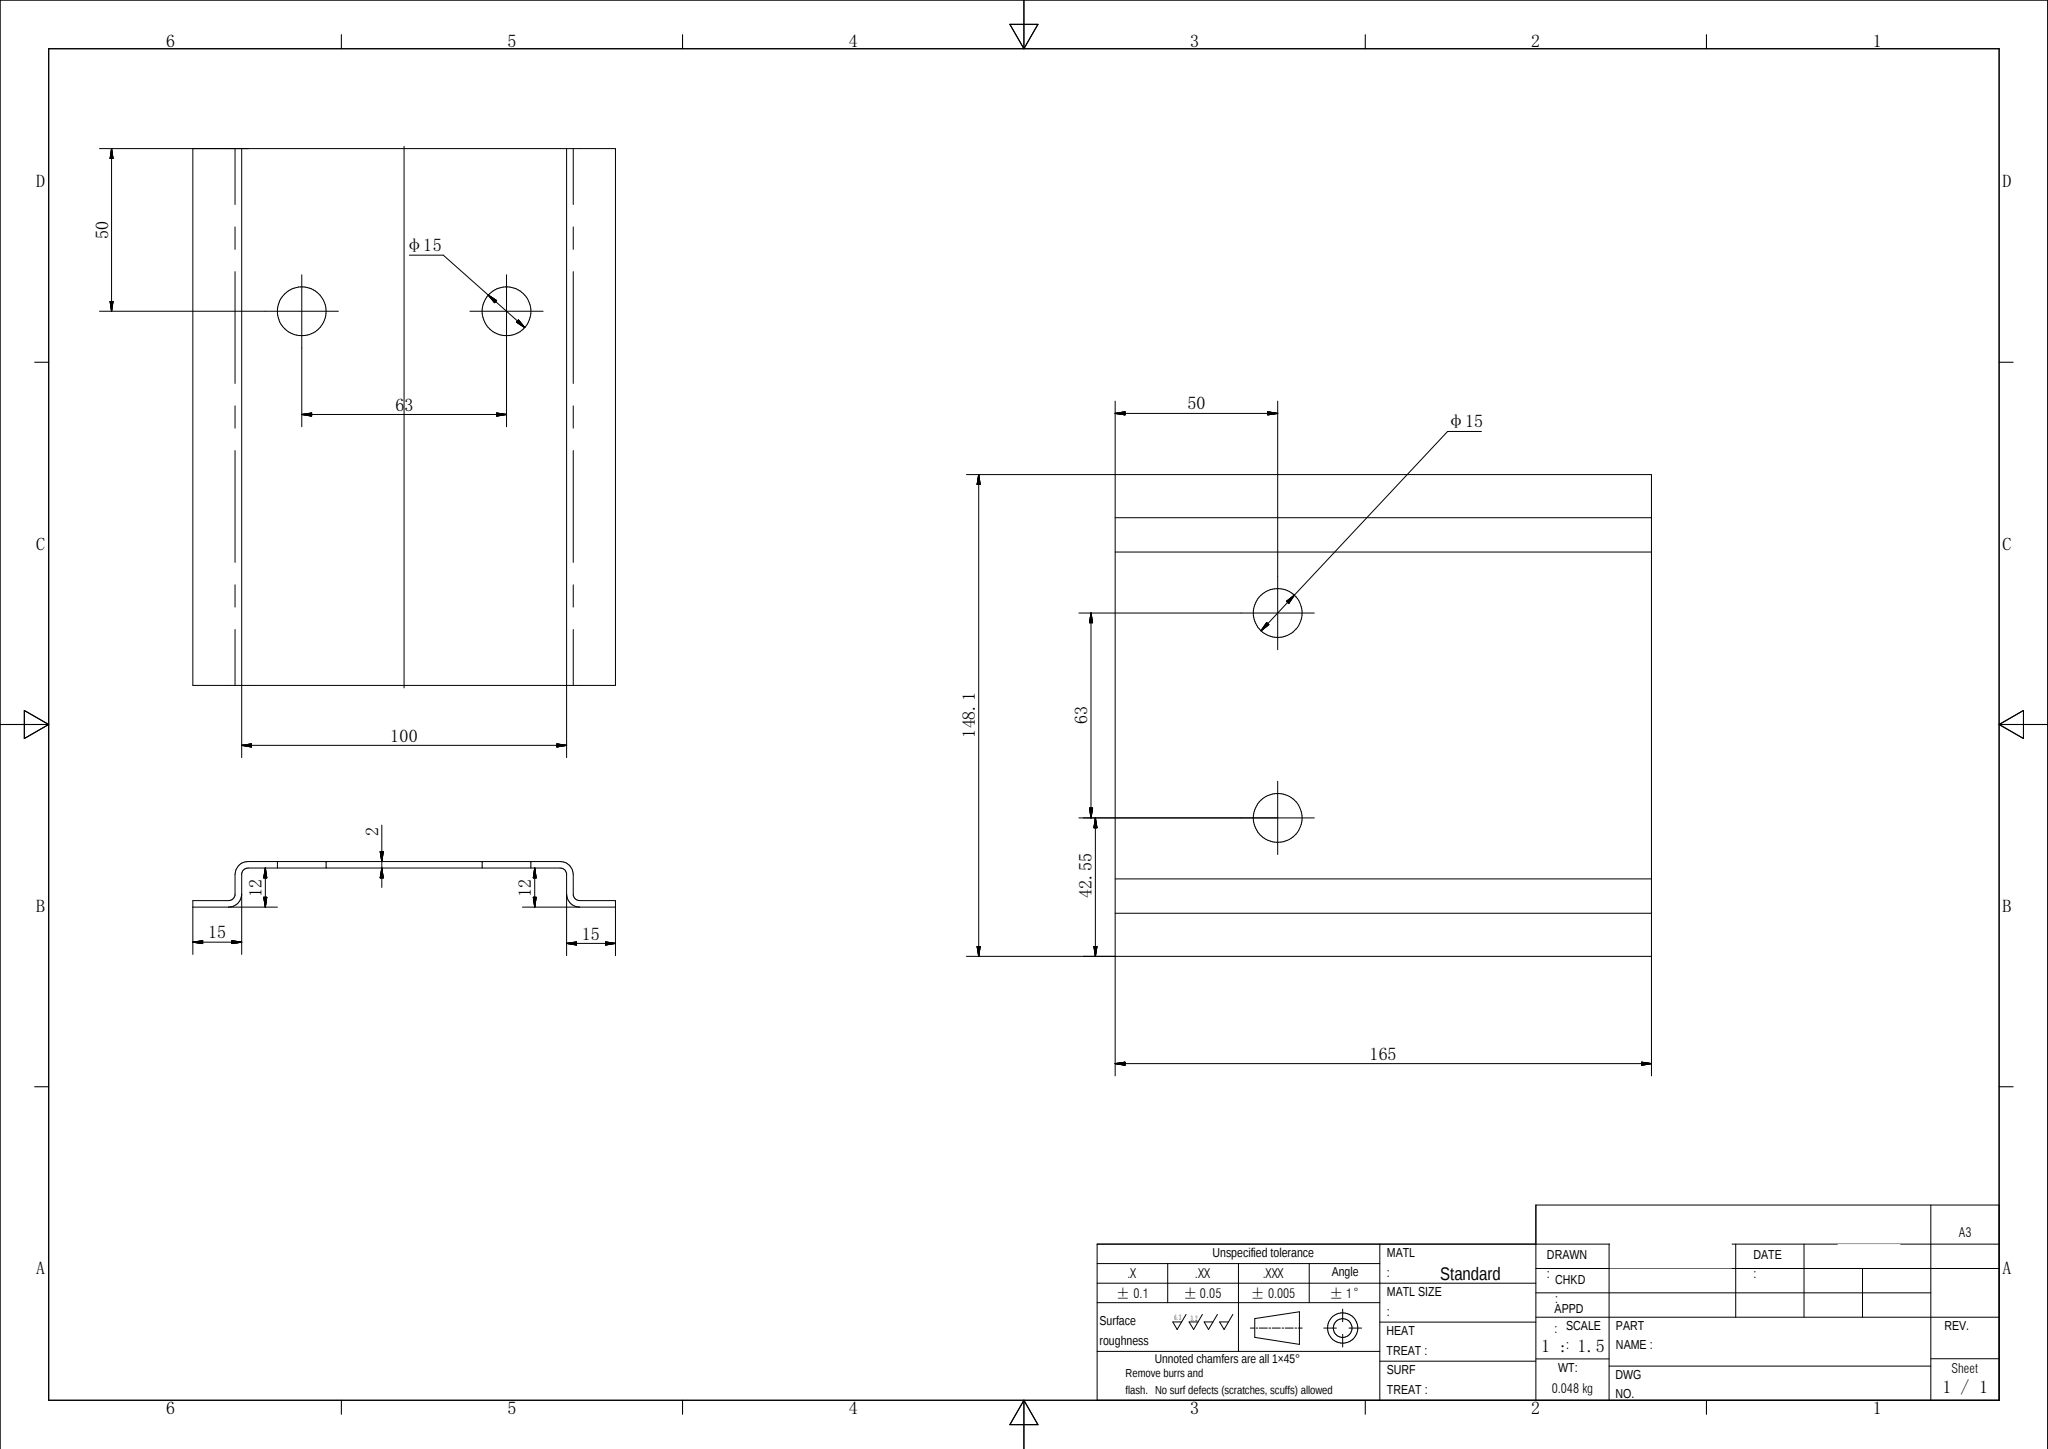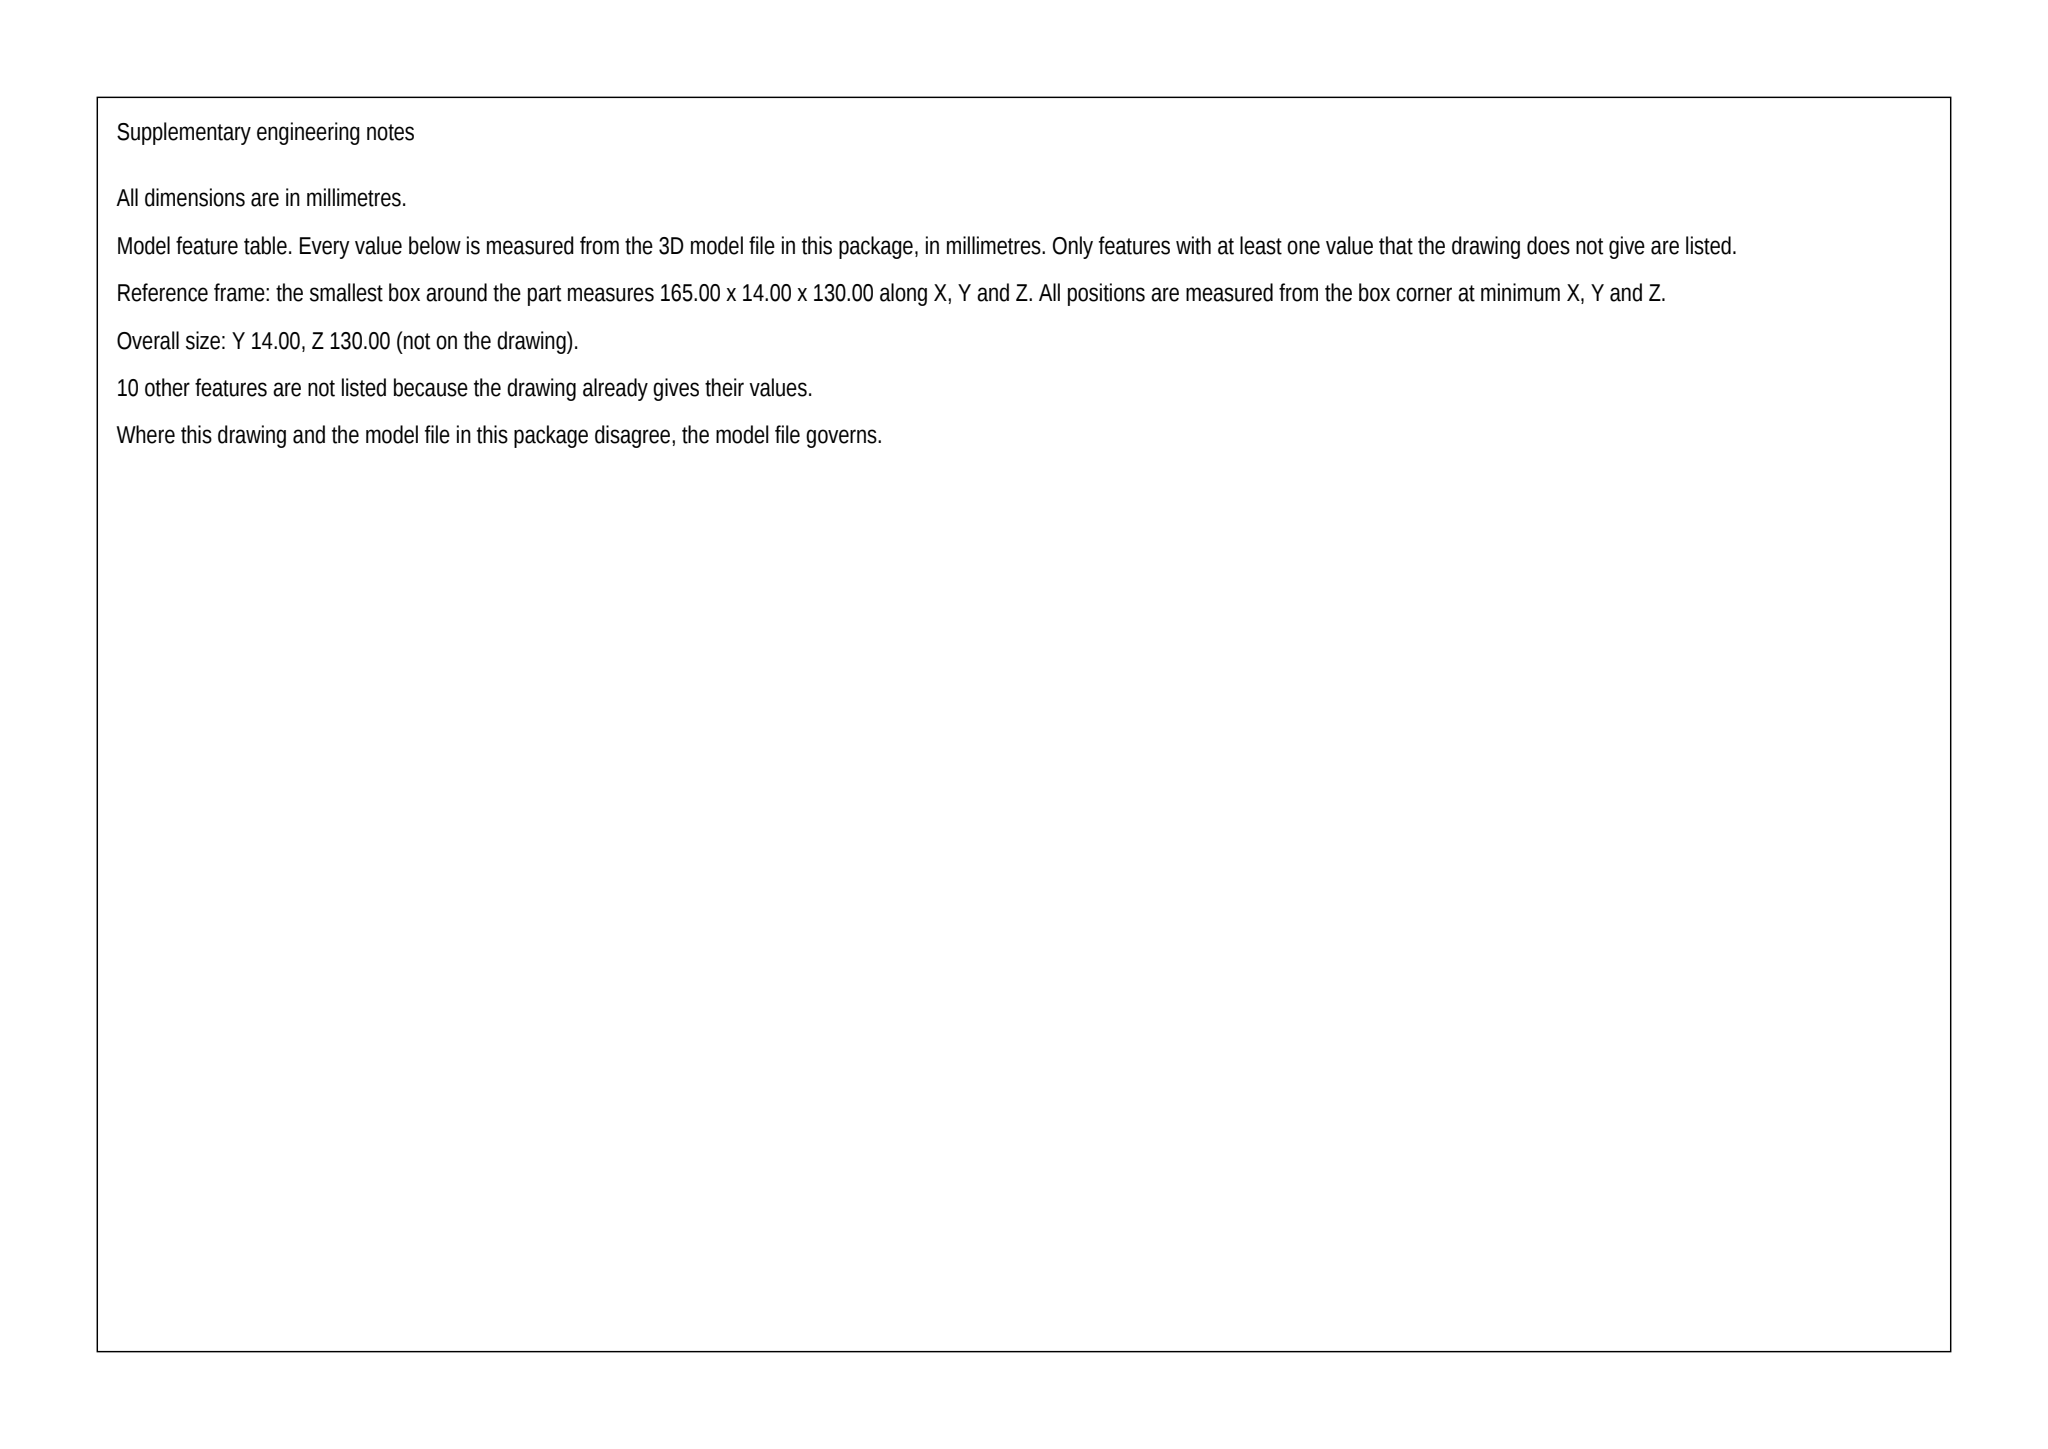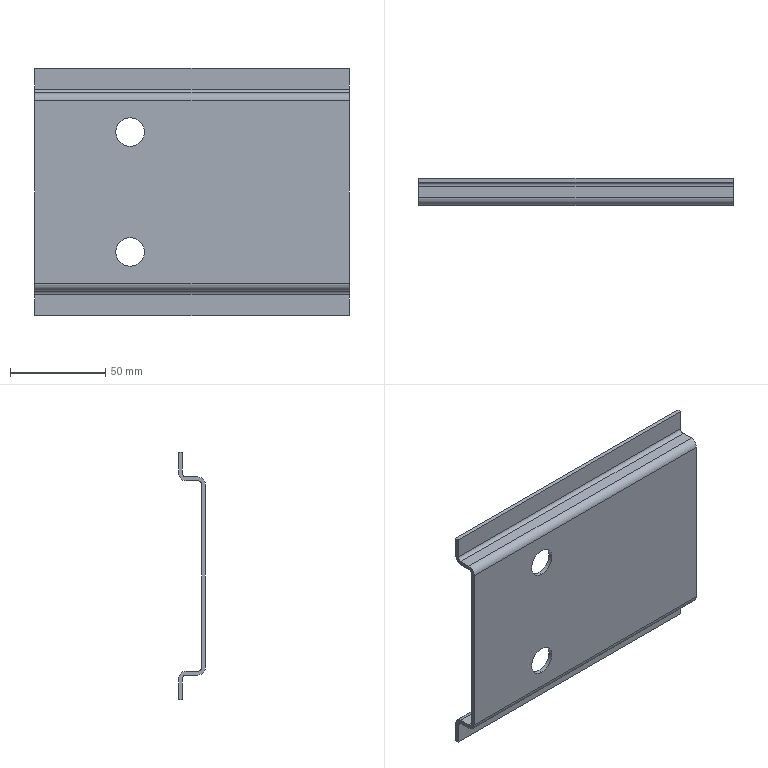Part | SolidWorks | mm | 1 solid | 26 faces | box 165 x 14 x 130 mm | volume 48413 mm3 | plane 14 | cylinder 12 | commonest cylinder face diameters 15 x4 4 x4 8 x4
Drawing notes:
ALL 4 BENDS: INSIDE R2, OUTSIDE R4 (THK 2) | from the solid: Cyl dia 4.0 (R2) and dia 8.0 (R4) along x at bend lines y=4/z=17,113 and y=10/z=11,119; plate planes y=0 & y=2 give THK 2
STEP:
#1=CARTESIAN_POINT('',(-32.5,0.,-39.));
#2=VERTEX_POINT('',#1);
#3=CARTESIAN_POINT('',(-32.5,0.,-24.));
#4=VERTEX_POINT('',#3);
#5=CARTESIAN_POINT('',(-32.5,0.,-31.5));
#6=DIRECTION('',(0.,1.,0.));
#7=DIRECTION('',(0.,0.,1.));
#8=AXIS2_PLACEMENT_3D('',#5,#6,#7);
#9=CIRCLE('',#8,7.5);
#10=EDGE_CURVE('',#2,#4,#9,.T.);
#11=ORIENTED_EDGE('',*,*,#10,.F.);
#12=CARTESIAN_POINT('',(-32.5,2.,-39.));
#13=VERTEX_POINT('',#12);
#14=CARTESIAN_POINT('',(-32.5,1.,-39.));
#15=DIRECTION('',(0.,1.,0.));
#16=VECTOR('',#15,1000.);
#17=LINE('',#14,#16);
#18=EDGE_CURVE('',#2,#13,#17,.T.);
#19=ORIENTED_EDGE('',*,*,#18,.T.);
#20=CARTESIAN_POINT('',(-32.5,2.,-24.));
#21=VERTEX_POINT('',#20);
#22=CARTESIAN_POINT('',(-32.5,2.,-31.5));
#23=DIRECTION('',(0.,-1.,0.));
#24=DIRECTION('',(0.,0.,1.));
#25=AXIS2_PLACEMENT_3D('',#22,#23,#24);
#26=CIRCLE('',#25,7.5);
#27=EDGE_CURVE('',#21,#13,#26,.T.);
#28=ORIENTED_EDGE('',*,*,#27,.F.);
#29=CARTESIAN_POINT('',(-32.5,1.,-24.));
#30=DIRECTION('',(0.,1.,0.));
#31=VECTOR('',#30,1000.);
#32=LINE('',#29,#31);
#33=EDGE_CURVE('',#4,#21,#32,.T.);
#34=ORIENTED_EDGE('',*,*,#33,.F.);
#35=EDGE_LOOP('',(#11,#19,#28,#34));
#36=FACE_OUTER_BOUND('',#35,.T.);
#37=CARTESIAN_POINT('',(-32.5,1.,-31.5));
#38=DIRECTION('',(0.,1.,0.));
#39=DIRECTION('',(0.,0.,1.));
#40=AXIS2_PLACEMENT_3D('',#37,#38,#39);
#41=CYLINDRICAL_SURFACE('',#40,7.5);
#42=ADVANCED_FACE('',(#36),#41,.F.);
#43=CARTESIAN_POINT('',(-32.5,0.,24.));
#44=VERTEX_POINT('',#43);
#45=CARTESIAN_POINT('',(-32.5,0.,39.));
#46=VERTEX_POINT('',#45);
#47=CARTESIAN_POINT('',(-32.5,0.,31.5));
#48=DIRECTION('',(0.,1.,0.));
#49=DIRECTION('',(0.,0.,1.));
#50=AXIS2_PLACEMENT_3D('',#47,#48,#49);
#51=CIRCLE('',#50,7.5);
#52=EDGE_CURVE('',#44,#46,#51,.T.);
#53=ORIENTED_EDGE('',*,*,#52,.F.);
#54=CARTESIAN_POINT('',(-32.5,2.,24.));
#55=VERTEX_POINT('',#54);
#56=CARTESIAN_POINT('',(-32.5,1.,24.));
#57=DIRECTION('',(0.,1.,0.));
#58=VECTOR('',#57,1000.);
#59=LINE('',#56,#58);
#60=EDGE_CURVE('',#44,#55,#59,.T.);
#61=ORIENTED_EDGE('',*,*,#60,.T.);
#62=CARTESIAN_POINT('',(-32.5,2.,39.));
#63=VERTEX_POINT('',#62);
#64=CARTESIAN_POINT('',(-32.5,2.,31.5));
#65=DIRECTION('',(0.,-1.,0.));
#66=DIRECTION('',(0.,0.,1.));
#67=AXIS2_PLACEMENT_3D('',#64,#65,#66);
#68=CIRCLE('',#67,7.5);
#69=EDGE_CURVE('',#63,#55,#68,.T.);
#70=ORIENTED_EDGE('',*,*,#69,.F.);
#71=CARTESIAN_POINT('',(-32.5,1.,39.));
#72=DIRECTION('',(0.,1.,0.));
#73=VECTOR('',#72,1000.);
#74=LINE('',#71,#73);
#75=EDGE_CURVE('',#46,#63,#74,.T.);
#76=ORIENTED_EDGE('',*,*,#75,.F.);
#77=EDGE_LOOP('',(#53,#61,#70,#76));
#78=FACE_OUTER_BOUND('',#77,.T.);
#79=CARTESIAN_POINT('',(-32.5,1.,31.5));
#80=DIRECTION('',(0.,1.,0.));
#81=DIRECTION('',(0.,0.,1.));
#82=AXIS2_PLACEMENT_3D('',#79,#80,#81);
#83=CYLINDRICAL_SURFACE('',#82,7.5);
#84=ADVANCED_FACE('',(#78),#83,.F.);
#85=ORIENTED_EDGE('',*,*,#27,.T.);
#86=CARTESIAN_POINT('',(-32.5,2.,-31.5));
#87=DIRECTION('',(0.,-1.,0.));
#88=DIRECTION('',(0.,0.,1.));
#89=AXIS2_PLACEMENT_3D('',#86,#87,#88);
#90=CIRCLE('',#89,7.5);
#91=EDGE_CURVE('',#13,#21,#90,.T.);
#92=ORIENTED_EDGE('',*,*,#91,.T.);
#93=EDGE_LOOP('',(#85,#92));
#94=FACE_BOUND('',#93,.T.);
#95=ORIENTED_EDGE('',*,*,#69,.T.);
#96=CARTESIAN_POINT('',(-32.5,2.,31.5));
#97=DIRECTION('',(0.,-1.,0.));
#98=DIRECTION('',(0.,0.,1.));
#99=AXIS2_PLACEMENT_3D('',#96,#97,#98);
#100=CIRCLE('',#99,7.5);
#101=EDGE_CURVE('',#55,#63,#100,.T.);
#102=ORIENTED_EDGE('',*,*,#101,.T.);
#103=EDGE_LOOP('',(#95,#102));
#104=FACE_BOUND('',#103,.T.);
#105=CARTESIAN_POINT('',(-82.5,2.,48.));
#106=VERTEX_POINT('',#105);
#107=CARTESIAN_POINT('',(82.5,2.,48.));
#108=VERTEX_POINT('',#107);
#109=CARTESIAN_POINT('',(-0.,2.,48.));
#110=DIRECTION('',(1.,0.,0.));
#111=VECTOR('',#110,1000.);
#112=LINE('',#109,#111);
#113=EDGE_CURVE('',#106,#108,#112,.T.);
#114=ORIENTED_EDGE('',*,*,#113,.T.);
#115=CARTESIAN_POINT('',(82.5,2.,-48.));
#116=VERTEX_POINT('',#115);
#117=CARTESIAN_POINT('',(82.5,2.,0.));
#118=DIRECTION('',(0.,0.,-1.));
#119=VECTOR('',#118,1000.);
#120=LINE('',#117,#119);
#121=EDGE_CURVE('',#108,#116,#120,.T.);
#122=ORIENTED_EDGE('',*,*,#121,.T.);
#123=CARTESIAN_POINT('',(-82.5,2.,-48.));
#124=VERTEX_POINT('',#123);
#125=CARTESIAN_POINT('',(-0.,2.,-48.));
#126=DIRECTION('',(-1.,0.,0.));
#127=VECTOR('',#126,1000.);
#128=LINE('',#125,#127);
#129=EDGE_CURVE('',#116,#124,#128,.T.);
#130=ORIENTED_EDGE('',*,*,#129,.T.);
#131=CARTESIAN_POINT('',(-82.5,2.,0.));
#132=DIRECTION('',(0.,0.,1.));
#133=VECTOR('',#132,1000.);
#134=LINE('',#131,#133);
#135=EDGE_CURVE('',#124,#106,#134,.T.);
#136=ORIENTED_EDGE('',*,*,#135,.T.);
#137=EDGE_LOOP('',(#114,#122,#130,#136));
#138=FACE_OUTER_BOUND('',#137,.T.);
#139=CARTESIAN_POINT('',(-0.,2.,0.));
#140=DIRECTION('',(0.,1.,0.));
#141=DIRECTION('',(0.,0.,1.));
#142=AXIS2_PLACEMENT_3D('',#139,#140,#141);
#143=PLANE('',#142);
#144=ADVANCED_FACE('',(#94,#104,#138),#143,.T.);
#145=ORIENTED_EDGE('',*,*,#18,.F.);
#146=CARTESIAN_POINT('',(-32.5,0.,-31.5));
#147=DIRECTION('',(0.,1.,0.));
#148=DIRECTION('',(0.,0.,1.));
#149=AXIS2_PLACEMENT_3D('',#146,#147,#148);
#150=CIRCLE('',#149,7.5);
#151=EDGE_CURVE('',#4,#2,#150,.T.);
#152=ORIENTED_EDGE('',*,*,#151,.F.);
#153=ORIENTED_EDGE('',*,*,#33,.T.);
#154=ORIENTED_EDGE('',*,*,#91,.F.);
#155=EDGE_LOOP('',(#145,#152,#153,#154));
#156=FACE_OUTER_BOUND('',#155,.T.);
#157=CARTESIAN_POINT('',(-32.5,1.,-31.5));
#158=DIRECTION('',(0.,1.,0.));
#159=DIRECTION('',(0.,0.,1.));
#160=AXIS2_PLACEMENT_3D('',#157,#158,#159);
#161=CYLINDRICAL_SURFACE('',#160,7.5);
#162=ADVANCED_FACE('',(#156),#161,.F.);
#163=ORIENTED_EDGE('',*,*,#60,.F.);
#164=CARTESIAN_POINT('',(-32.5,0.,31.5));
#165=DIRECTION('',(0.,1.,0.));
#166=DIRECTION('',(0.,0.,1.));
#167=AXIS2_PLACEMENT_3D('',#164,#165,#166);
#168=CIRCLE('',#167,7.5);
#169=EDGE_CURVE('',#46,#44,#168,.T.);
#170=ORIENTED_EDGE('',*,*,#169,.F.);
#171=ORIENTED_EDGE('',*,*,#75,.T.);
#172=ORIENTED_EDGE('',*,*,#101,.F.);
#173=EDGE_LOOP('',(#163,#170,#171,#172));
#174=FACE_OUTER_BOUND('',#173,.T.);
#175=CARTESIAN_POINT('',(-32.5,1.,31.5));
#176=DIRECTION('',(0.,1.,0.));
#177=DIRECTION('',(0.,0.,1.));
#178=AXIS2_PLACEMENT_3D('',#175,#176,#177);
#179=CYLINDRICAL_SURFACE('',#178,7.5);
#180=ADVANCED_FACE('',(#174),#179,.F.);
#181=ORIENTED_EDGE('',*,*,#121,.F.);
#182=CARTESIAN_POINT('',(82.5,4.,50.));
#183=VERTEX_POINT('',#182);
#184=CARTESIAN_POINT('',(82.5,4.,48.));
#185=DIRECTION('',(-1.,0.,0.));
#186=DIRECTION('',(0.,0.,1.));
#187=AXIS2_PLACEMENT_3D('',#184,#185,#186);
#188=CIRCLE('',#187,2.);
#189=EDGE_CURVE('',#108,#183,#188,.T.);
#190=ORIENTED_EDGE('',*,*,#189,.T.);
#191=CARTESIAN_POINT('',(82.5,10.,50.));
#192=VERTEX_POINT('',#191);
#193=CARTESIAN_POINT('',(82.5,6.738,50.));
#194=DIRECTION('',(0.,-1.,-0.));
#195=VECTOR('',#194,1000.);
#196=LINE('',#193,#195);
#197=EDGE_CURVE('',#192,#183,#196,.T.);
#198=ORIENTED_EDGE('',*,*,#197,.F.);
#199=CARTESIAN_POINT('',(82.5,14.,54.));
#200=VERTEX_POINT('',#199);
#201=CARTESIAN_POINT('',(82.5,10.,54.));
#202=DIRECTION('',(-1.,0.,0.));
#203=DIRECTION('',(0.,-0.,-1.));
#204=AXIS2_PLACEMENT_3D('',#201,#202,#203);
#205=CIRCLE('',#204,4.);
#206=EDGE_CURVE('',#200,#192,#205,.T.);
#207=ORIENTED_EDGE('',*,*,#206,.F.);
#208=CARTESIAN_POINT('',(82.5,14.,65.));
#209=VERTEX_POINT('',#208);
#210=CARTESIAN_POINT('',(82.5,14.,57.238));
#211=DIRECTION('',(0.,-0.,1.));
#212=VECTOR('',#211,1000.);
#213=LINE('',#210,#212);
#214=EDGE_CURVE('',#200,#209,#213,.T.);
#215=ORIENTED_EDGE('',*,*,#214,.T.);
#216=CARTESIAN_POINT('',(82.5,12.,65.));
#217=VERTEX_POINT('',#216);
#218=CARTESIAN_POINT('',(82.5,12.,65.));
#219=DIRECTION('',(-0.,-1.,0.));
#220=VECTOR('',#219,1000.);
#221=LINE('',#218,#220);
#222=EDGE_CURVE('',#209,#217,#221,.T.);
#223=ORIENTED_EDGE('',*,*,#222,.T.);
#224=CARTESIAN_POINT('',(82.5,12.,54.));
#225=VERTEX_POINT('',#224);
#226=CARTESIAN_POINT('',(82.5,12.,54.));
#227=DIRECTION('',(0.,-0.,-1.));
#228=VECTOR('',#227,1000.);
#229=LINE('',#226,#228);
#230=EDGE_CURVE('',#217,#225,#229,.T.);
#231=ORIENTED_EDGE('',*,*,#230,.T.);
#232=CARTESIAN_POINT('',(82.5,10.,52.));
#233=VERTEX_POINT('',#232);
#234=CARTESIAN_POINT('',(82.5,10.,54.));
#235=DIRECTION('',(-1.,0.,0.));
#236=DIRECTION('',(0.,-0.,-1.));
#237=AXIS2_PLACEMENT_3D('',#234,#235,#236);
#238=CIRCLE('',#237,2.);
#239=EDGE_CURVE('',#225,#233,#238,.T.);
#240=ORIENTED_EDGE('',*,*,#239,.T.);
#241=CARTESIAN_POINT('',(82.5,4.,52.));
#242=VERTEX_POINT('',#241);
#243=CARTESIAN_POINT('',(82.5,4.,52.));
#244=DIRECTION('',(0.,-1.,-0.));
#245=VECTOR('',#244,1000.);
#246=LINE('',#243,#245);
#247=EDGE_CURVE('',#233,#242,#246,.T.);
#248=ORIENTED_EDGE('',*,*,#247,.T.);
#249=CARTESIAN_POINT('',(82.5,0.,48.));
#250=VERTEX_POINT('',#249);
#251=CARTESIAN_POINT('',(82.5,4.,48.));
#252=DIRECTION('',(1.,0.,-0.));
#253=DIRECTION('',(0.,-0.,1.));
#254=AXIS2_PLACEMENT_3D('',#251,#252,#253);
#255=CIRCLE('',#254,4.);
#256=EDGE_CURVE('',#242,#250,#255,.T.);
#257=ORIENTED_EDGE('',*,*,#256,.T.);
#258=CARTESIAN_POINT('',(82.5,0.,-48.));
#259=VERTEX_POINT('',#258);
#260=CARTESIAN_POINT('',(82.5,0.,-52.));
#261=DIRECTION('',(0.,0.,-1.));
#262=VECTOR('',#261,1000.);
#263=LINE('',#260,#262);
#264=EDGE_CURVE('',#250,#259,#263,.T.);
#265=ORIENTED_EDGE('',*,*,#264,.T.);
#266=CARTESIAN_POINT('',(82.5,4.,-52.));
#267=VERTEX_POINT('',#266);
#268=CARTESIAN_POINT('',(82.5,4.,-48.));
#269=DIRECTION('',(1.,0.,0.));
#270=DIRECTION('',(0.,0.,-1.));
#271=AXIS2_PLACEMENT_3D('',#268,#269,#270);
#272=CIRCLE('',#271,4.);
#273=EDGE_CURVE('',#259,#267,#272,.T.);
#274=ORIENTED_EDGE('',*,*,#273,.T.);
#275=CARTESIAN_POINT('',(82.5,10.,-52.));
#276=VERTEX_POINT('',#275);
#277=CARTESIAN_POINT('',(82.5,4.,-52.));
#278=DIRECTION('',(0.,1.,0.));
#279=VECTOR('',#278,1000.);
#280=LINE('',#277,#279);
#281=EDGE_CURVE('',#267,#276,#280,.T.);
#282=ORIENTED_EDGE('',*,*,#281,.T.);
#283=CARTESIAN_POINT('',(82.5,12.,-54.));
#284=VERTEX_POINT('',#283);
#285=CARTESIAN_POINT('',(82.5,10.,-54.));
#286=DIRECTION('',(-1.,0.,-0.));
#287=DIRECTION('',(0.,0.,1.));
#288=AXIS2_PLACEMENT_3D('',#285,#286,#287);
#289=CIRCLE('',#288,2.);
#290=EDGE_CURVE('',#276,#284,#289,.T.);
#291=ORIENTED_EDGE('',*,*,#290,.T.);
#292=CARTESIAN_POINT('',(82.5,12.,-65.));
#293=VERTEX_POINT('',#292);
#294=CARTESIAN_POINT('',(82.5,12.,-54.));
#295=DIRECTION('',(0.,-0.,-1.));
#296=VECTOR('',#295,1000.);
#297=LINE('',#294,#296);
#298=EDGE_CURVE('',#284,#293,#297,.T.);
#299=ORIENTED_EDGE('',*,*,#298,.T.);
#300=CARTESIAN_POINT('',(82.5,14.,-65.));
#301=VERTEX_POINT('',#300);
#302=CARTESIAN_POINT('',(82.5,12.,-65.));
#303=DIRECTION('',(0.,1.,0.));
#304=VECTOR('',#303,1000.);
#305=LINE('',#302,#304);
#306=EDGE_CURVE('',#293,#301,#305,.T.);
#307=ORIENTED_EDGE('',*,*,#306,.T.);
#308=CARTESIAN_POINT('',(82.5,14.,-54.));
#309=VERTEX_POINT('',#308);
#310=CARTESIAN_POINT('',(82.5,14.,-57.238));
#311=DIRECTION('',(0.,0.,-1.));
#312=VECTOR('',#311,1000.);
#313=LINE('',#310,#312);
#314=EDGE_CURVE('',#309,#301,#313,.T.);
#315=ORIENTED_EDGE('',*,*,#314,.F.);
#316=CARTESIAN_POINT('',(82.5,10.,-50.));
#317=VERTEX_POINT('',#316);
#318=CARTESIAN_POINT('',(82.5,10.,-54.));
#319=DIRECTION('',(-1.,0.,-0.));
#320=DIRECTION('',(0.,0.,1.));
#321=AXIS2_PLACEMENT_3D('',#318,#319,#320);
#322=CIRCLE('',#321,4.);
#323=EDGE_CURVE('',#317,#309,#322,.T.);
#324=ORIENTED_EDGE('',*,*,#323,.F.);
#325=CARTESIAN_POINT('',(82.5,4.,-50.));
#326=VERTEX_POINT('',#325);
#327=CARTESIAN_POINT('',(82.5,6.738,-50.));
#328=DIRECTION('',(0.,1.,0.));
#329=VECTOR('',#328,1000.);
#330=LINE('',#327,#329);
#331=EDGE_CURVE('',#326,#317,#330,.T.);
#332=ORIENTED_EDGE('',*,*,#331,.F.);
#333=CARTESIAN_POINT('',(82.5,4.,-48.));
#334=DIRECTION('',(-1.,0.,0.));
#335=DIRECTION('',(0.,0.,-1.));
#336=AXIS2_PLACEMENT_3D('',#333,#334,#335);
#337=CIRCLE('',#336,2.);
#338=EDGE_CURVE('',#326,#116,#337,.T.);
#339=ORIENTED_EDGE('',*,*,#338,.T.);
#340=EDGE_LOOP('',(#181,#190,#198,#207,#215,#223,#231,#240,#248,#257,#265,#274,#282,#291,#299,#307,#315,#324,#332,#339));
#341=FACE_OUTER_BOUND('',#340,.T.);
#342=CARTESIAN_POINT('',(82.5,0.,-52.));
#343=DIRECTION('',(1.,0.,0.));
#344=DIRECTION('',(0.,0.,-1.));
#345=AXIS2_PLACEMENT_3D('',#342,#343,#344);
#346=PLANE('',#345);
#347=ADVANCED_FACE('',(#341),#346,.T.);
#348=ORIENTED_EDGE('',*,*,#189,.F.);
#349=ORIENTED_EDGE('',*,*,#113,.F.);
#350=CARTESIAN_POINT('',(-82.5,4.,50.));
#351=VERTEX_POINT('',#350);
#352=CARTESIAN_POINT('',(-82.5,4.,48.));
#353=DIRECTION('',(1.,0.,-0.));
#354=DIRECTION('',(0.,-0.,1.));
#355=AXIS2_PLACEMENT_3D('',#352,#353,#354);
#356=CIRCLE('',#355,2.);
#357=EDGE_CURVE('',#351,#106,#356,.T.);
#358=ORIENTED_EDGE('',*,*,#357,.F.);
#359=CARTESIAN_POINT('',(0.,4.,50.));
#360=DIRECTION('',(-1.,0.,0.));
#361=VECTOR('',#360,1000.);
#362=LINE('',#359,#361);
#363=EDGE_CURVE('',#183,#351,#362,.T.);
#364=ORIENTED_EDGE('',*,*,#363,.F.);
#365=EDGE_LOOP('',(#348,#349,#358,#364));
#366=FACE_OUTER_BOUND('',#365,.T.);
#367=CARTESIAN_POINT('',(0.,4.,48.));
#368=DIRECTION('',(-1.,0.,0.));
#369=DIRECTION('',(0.,0.,1.));
#370=AXIS2_PLACEMENT_3D('',#367,#368,#369);
#371=CYLINDRICAL_SURFACE('',#370,2.);
#372=ADVANCED_FACE('',(#366),#371,.F.);
#373=CARTESIAN_POINT('',(-82.5,0.,-48.));
#374=VERTEX_POINT('',#373);
#375=CARTESIAN_POINT('',(-82.5,0.,48.));
#376=VERTEX_POINT('',#375);
#377=CARTESIAN_POINT('',(-82.5,0.,52.));
#378=DIRECTION('',(0.,0.,1.));
#379=VECTOR('',#378,1000.);
#380=LINE('',#377,#379);
#381=EDGE_CURVE('',#374,#376,#380,.T.);
#382=ORIENTED_EDGE('',*,*,#381,.T.);
#383=CARTESIAN_POINT('',(-82.5,4.,52.));
#384=VERTEX_POINT('',#383);
#385=CARTESIAN_POINT('',(-82.5,4.,48.));
#386=DIRECTION('',(-1.,0.,0.));
#387=DIRECTION('',(0.,0.,1.));
#388=AXIS2_PLACEMENT_3D('',#385,#386,#387);
#389=CIRCLE('',#388,4.);
#390=EDGE_CURVE('',#376,#384,#389,.T.);
#391=ORIENTED_EDGE('',*,*,#390,.T.);
#392=CARTESIAN_POINT('',(-82.5,10.,52.));
#393=VERTEX_POINT('',#392);
#394=CARTESIAN_POINT('',(-82.5,4.,52.));
#395=DIRECTION('',(0.,1.,0.));
#396=VECTOR('',#395,1000.);
#397=LINE('',#394,#396);
#398=EDGE_CURVE('',#384,#393,#397,.T.);
#399=ORIENTED_EDGE('',*,*,#398,.T.);
#400=CARTESIAN_POINT('',(-82.5,12.,54.));
#401=VERTEX_POINT('',#400);
#402=CARTESIAN_POINT('',(-82.5,10.,54.));
#403=DIRECTION('',(1.,-0.,-0.));
#404=DIRECTION('',(0.,0.,-1.));
#405=AXIS2_PLACEMENT_3D('',#402,#403,#404);
#406=CIRCLE('',#405,2.);
#407=EDGE_CURVE('',#393,#401,#406,.T.);
#408=ORIENTED_EDGE('',*,*,#407,.T.);
#409=CARTESIAN_POINT('',(-82.5,12.,65.));
#410=VERTEX_POINT('',#409);
#411=CARTESIAN_POINT('',(-82.5,12.,54.));
#412=DIRECTION('',(0.,0.,1.));
#413=VECTOR('',#412,1000.);
#414=LINE('',#411,#413);
#415=EDGE_CURVE('',#401,#410,#414,.T.);
#416=ORIENTED_EDGE('',*,*,#415,.T.);
#417=CARTESIAN_POINT('',(-82.5,14.,65.));
#418=VERTEX_POINT('',#417);
#419=CARTESIAN_POINT('',(-82.5,12.,65.));
#420=DIRECTION('',(0.,1.,-0.));
#421=VECTOR('',#420,1000.);
#422=LINE('',#419,#421);
#423=EDGE_CURVE('',#410,#418,#422,.T.);
#424=ORIENTED_EDGE('',*,*,#423,.T.);
#425=CARTESIAN_POINT('',(-82.5,14.,54.));
#426=VERTEX_POINT('',#425);
#427=CARTESIAN_POINT('',(-82.5,14.,57.238));
#428=DIRECTION('',(0.,0.,-1.));
#429=VECTOR('',#428,1000.);
#430=LINE('',#427,#429);
#431=EDGE_CURVE('',#418,#426,#430,.T.);
#432=ORIENTED_EDGE('',*,*,#431,.T.);
#433=CARTESIAN_POINT('',(-82.5,10.,50.));
#434=VERTEX_POINT('',#433);
#435=CARTESIAN_POINT('',(-82.5,10.,54.));
#436=DIRECTION('',(1.,-0.,-0.));
#437=DIRECTION('',(0.,0.,-1.));
#438=AXIS2_PLACEMENT_3D('',#435,#436,#437);
#439=CIRCLE('',#438,4.);
#440=EDGE_CURVE('',#434,#426,#439,.T.);
#441=ORIENTED_EDGE('',*,*,#440,.F.);
#442=CARTESIAN_POINT('',(-82.5,6.738,50.));
#443=DIRECTION('',(0.,1.,0.));
#444=VECTOR('',#443,1000.);
#445=LINE('',#442,#444);
#446=EDGE_CURVE('',#351,#434,#445,.T.);
#447=ORIENTED_EDGE('',*,*,#446,.F.);
#448=ORIENTED_EDGE('',*,*,#357,.T.);
#449=ORIENTED_EDGE('',*,*,#135,.F.);
#450=CARTESIAN_POINT('',(-82.5,4.,-50.));
#451=VERTEX_POINT('',#450);
#452=CARTESIAN_POINT('',(-82.5,4.,-48.));
#453=DIRECTION('',(1.,0.,0.));
#454=DIRECTION('',(0.,0.,-1.));
#455=AXIS2_PLACEMENT_3D('',#452,#453,#454);
#456=CIRCLE('',#455,2.);
#457=EDGE_CURVE('',#124,#451,#456,.T.);
#458=ORIENTED_EDGE('',*,*,#457,.T.);
#459=CARTESIAN_POINT('',(-82.5,10.,-50.));
#460=VERTEX_POINT('',#459);
#461=CARTESIAN_POINT('',(-82.5,6.738,-50.));
#462=DIRECTION('',(0.,-1.,-0.));
#463=VECTOR('',#462,1000.);
#464=LINE('',#461,#463);
#465=EDGE_CURVE('',#460,#451,#464,.T.);
#466=ORIENTED_EDGE('',*,*,#465,.F.);
#467=CARTESIAN_POINT('',(-82.5,14.,-54.));
#468=VERTEX_POINT('',#467);
#469=CARTESIAN_POINT('',(-82.5,10.,-54.));
#470=DIRECTION('',(1.,-0.,0.));
#471=DIRECTION('',(0.,0.,1.));
#472=AXIS2_PLACEMENT_3D('',#469,#470,#471);
#473=CIRCLE('',#472,4.);
#474=EDGE_CURVE('',#468,#460,#473,.T.);
#475=ORIENTED_EDGE('',*,*,#474,.F.);
#476=CARTESIAN_POINT('',(-82.5,14.,-65.));
#477=VERTEX_POINT('',#476);
#478=CARTESIAN_POINT('',(-82.5,14.,-57.238));
#479=DIRECTION('',(0.,-0.,1.));
#480=VECTOR('',#479,1000.);
#481=LINE('',#478,#480);
#482=EDGE_CURVE('',#477,#468,#481,.T.);
#483=ORIENTED_EDGE('',*,*,#482,.F.);
#484=CARTESIAN_POINT('',(-82.5,12.,-65.));
#485=VERTEX_POINT('',#484);
#486=CARTESIAN_POINT('',(-82.5,12.,-65.));
#487=DIRECTION('',(-0.,-1.,0.));
#488=VECTOR('',#487,1000.);
#489=LINE('',#486,#488);
#490=EDGE_CURVE('',#477,#485,#489,.T.);
#491=ORIENTED_EDGE('',*,*,#490,.T.);
#492=CARTESIAN_POINT('',(-82.5,12.,-54.));
#493=VERTEX_POINT('',#492);
#494=CARTESIAN_POINT('',(-82.5,12.,-54.));
#495=DIRECTION('',(-0.,0.,1.));
#496=VECTOR('',#495,1000.);
#497=LINE('',#494,#496);
#498=EDGE_CURVE('',#485,#493,#497,.T.);
#499=ORIENTED_EDGE('',*,*,#498,.T.);
#500=CARTESIAN_POINT('',(-82.5,10.,-52.));
#501=VERTEX_POINT('',#500);
#502=CARTESIAN_POINT('',(-82.5,10.,-54.));
#503=DIRECTION('',(1.,-0.,0.));
#504=DIRECTION('',(0.,0.,1.));
#505=AXIS2_PLACEMENT_3D('',#502,#503,#504);
#506=CIRCLE('',#505,2.);
#507=EDGE_CURVE('',#493,#501,#506,.T.);
#508=ORIENTED_EDGE('',*,*,#507,.T.);
#509=CARTESIAN_POINT('',(-82.5,4.,-52.));
#510=VERTEX_POINT('',#509);
#511=CARTESIAN_POINT('',(-82.5,4.,-52.));
#512=DIRECTION('',(0.,-1.,0.));
#513=VECTOR('',#512,1000.);
#514=LINE('',#511,#513);
#515=EDGE_CURVE('',#501,#510,#514,.T.);
#516=ORIENTED_EDGE('',*,*,#515,.T.);
#517=CARTESIAN_POINT('',(-82.5,4.,-48.));
#518=DIRECTION('',(-1.,0.,0.));
#519=DIRECTION('',(0.,0.,-1.));
#520=AXIS2_PLACEMENT_3D('',#517,#518,#519);
#521=CIRCLE('',#520,4.);
#522=EDGE_CURVE('',#510,#374,#521,.T.);
#523=ORIENTED_EDGE('',*,*,#522,.T.);
#524=EDGE_LOOP('',(#382,#391,#399,#408,#416,#424,#432,#441,#447,#448,#449,#458,#466,#475,#483,#491,#499,#508,#516,#523));
#525=FACE_OUTER_BOUND('',#524,.T.);
#526=CARTESIAN_POINT('',(-82.5,0.,52.));
#527=DIRECTION('',(-1.,0.,0.));
#528=DIRECTION('',(0.,0.,1.));
#529=AXIS2_PLACEMENT_3D('',#526,#527,#528);
#530=PLANE('',#529);
#531=ADVANCED_FACE('',(#525),#530,.T.);
#532=ORIENTED_EDGE('',*,*,#457,.F.);
#533=ORIENTED_EDGE('',*,*,#129,.F.);
#534=ORIENTED_EDGE('',*,*,#338,.F.);
#535=CARTESIAN_POINT('',(0.,4.,-50.));
#536=DIRECTION('',(1.,0.,0.));
#537=VECTOR('',#536,1000.);
#538=LINE('',#535,#537);
#539=EDGE_CURVE('',#451,#326,#538,.T.);
#540=ORIENTED_EDGE('',*,*,#539,.F.);
#541=EDGE_LOOP('',(#532,#533,#534,#540));
#542=FACE_OUTER_BOUND('',#541,.T.);
#543=CARTESIAN_POINT('',(0.,4.,-48.));
#544=DIRECTION('',(1.,0.,0.));
#545=DIRECTION('',(0.,0.,-1.));
#546=AXIS2_PLACEMENT_3D('',#543,#544,#545);
#547=CYLINDRICAL_SURFACE('',#546,2.);
#548=ADVANCED_FACE('',(#542),#547,.F.);
#549=ORIENTED_EDGE('',*,*,#151,.T.);
#550=ORIENTED_EDGE('',*,*,#10,.T.);
#551=EDGE_LOOP('',(#549,#550));
#552=FACE_BOUND('',#551,.T.);
#553=ORIENTED_EDGE('',*,*,#169,.T.);
#554=ORIENTED_EDGE('',*,*,#52,.T.);
#555=EDGE_LOOP('',(#553,#554));
#556=FACE_BOUND('',#555,.T.);
#557=ORIENTED_EDGE('',*,*,#264,.F.);
#558=CARTESIAN_POINT('',(-0.,0.,48.));
#559=DIRECTION('',(1.,0.,0.));
#560=VECTOR('',#559,1000.);
#561=LINE('',#558,#560);
#562=EDGE_CURVE('',#376,#250,#561,.T.);
#563=ORIENTED_EDGE('',*,*,#562,.F.);
#564=ORIENTED_EDGE('',*,*,#381,.F.);
#565=CARTESIAN_POINT('',(-0.,0.,-48.));
#566=DIRECTION('',(-1.,0.,0.));
#567=VECTOR('',#566,1000.);
#568=LINE('',#565,#567);
#569=EDGE_CURVE('',#259,#374,#568,.T.);
#570=ORIENTED_EDGE('',*,*,#569,.F.);
#571=EDGE_LOOP('',(#557,#563,#564,#570));
#572=FACE_OUTER_BOUND('',#571,.T.);
#573=CARTESIAN_POINT('',(-0.,0.,0.));
#574=DIRECTION('',(0.,1.,0.));
#575=DIRECTION('',(0.,0.,1.));
#576=AXIS2_PLACEMENT_3D('',#573,#574,#575);
#577=PLANE('',#576);
#578=ADVANCED_FACE('',(#552,#556,#572),#577,.F.);
#579=ORIENTED_EDGE('',*,*,#363,.T.);
#580=ORIENTED_EDGE('',*,*,#446,.T.);
#581=CARTESIAN_POINT('',(-0.,10.,50.));
#582=DIRECTION('',(1.,0.,-0.));
#583=VECTOR('',#582,1000.);
#584=LINE('',#581,#583);
#585=EDGE_CURVE('',#434,#192,#584,.T.);
#586=ORIENTED_EDGE('',*,*,#585,.T.);
#587=ORIENTED_EDGE('',*,*,#197,.T.);
#588=EDGE_LOOP('',(#579,#580,#586,#587));
#589=FACE_OUTER_BOUND('',#588,.T.);
#590=CARTESIAN_POINT('',(-0.,6.738,50.));
#591=DIRECTION('',(-0.,0.,-1.));
#592=DIRECTION('',(0.,1.,0.));
#593=AXIS2_PLACEMENT_3D('',#590,#591,#592);
#594=PLANE('',#593);
#595=ADVANCED_FACE('',(#589),#594,.T.);
#596=ORIENTED_EDGE('',*,*,#539,.T.);
#597=ORIENTED_EDGE('',*,*,#331,.T.);
#598=CARTESIAN_POINT('',(0.,10.,-50.));
#599=DIRECTION('',(-1.,-0.,0.));
#600=VECTOR('',#599,1000.);
#601=LINE('',#598,#600);
#602=EDGE_CURVE('',#317,#460,#601,.T.);
#603=ORIENTED_EDGE('',*,*,#602,.T.);
#604=ORIENTED_EDGE('',*,*,#465,.T.);
#605=EDGE_LOOP('',(#596,#597,#603,#604));
#606=FACE_OUTER_BOUND('',#605,.T.);
#607=CARTESIAN_POINT('',(0.,6.738,-50.));
#608=DIRECTION('',(0.,-0.,1.));
#609=DIRECTION('',(0.,-1.,-0.));
#610=AXIS2_PLACEMENT_3D('',#607,#608,#609);
#611=PLANE('',#610);
#612=ADVANCED_FACE('',(#606),#611,.T.);
#613=ORIENTED_EDGE('',*,*,#569,.T.);
#614=ORIENTED_EDGE('',*,*,#522,.F.);
#615=CARTESIAN_POINT('',(0.,4.,-52.));
#616=DIRECTION('',(1.,0.,0.));
#617=VECTOR('',#616,1000.);
#618=LINE('',#615,#617);
#619=EDGE_CURVE('',#510,#267,#618,.T.);
#620=ORIENTED_EDGE('',*,*,#619,.T.);
#621=ORIENTED_EDGE('',*,*,#273,.F.);
#622=EDGE_LOOP('',(#613,#614,#620,#621));
#623=FACE_OUTER_BOUND('',#622,.T.);
#624=CARTESIAN_POINT('',(0.,4.,-48.));
#625=DIRECTION('',(1.,0.,0.));
#626=DIRECTION('',(0.,0.,-1.));
#627=AXIS2_PLACEMENT_3D('',#624,#625,#626);
#628=CYLINDRICAL_SURFACE('',#627,4.);
#629=ADVANCED_FACE('',(#623),#628,.T.);
#630=ORIENTED_EDGE('',*,*,#562,.T.);
#631=ORIENTED_EDGE('',*,*,#256,.F.);
#632=CARTESIAN_POINT('',(0.,4.,52.));
#633=DIRECTION('',(-1.,0.,0.));
#634=VECTOR('',#633,1000.);
#635=LINE('',#632,#634);
#636=EDGE_CURVE('',#242,#384,#635,.T.);
#637=ORIENTED_EDGE('',*,*,#636,.T.);
#638=ORIENTED_EDGE('',*,*,#390,.F.);
#639=EDGE_LOOP('',(#630,#631,#637,#638));
#640=FACE_OUTER_BOUND('',#639,.T.);
#641=CARTESIAN_POINT('',(0.,4.,48.));
#642=DIRECTION('',(-1.,0.,0.));
#643=DIRECTION('',(0.,0.,1.));
#644=AXIS2_PLACEMENT_3D('',#641,#642,#643);
#645=CYLINDRICAL_SURFACE('',#644,4.);
#646=ADVANCED_FACE('',(#640),#645,.T.);
#647=ORIENTED_EDGE('',*,*,#585,.F.);
#648=ORIENTED_EDGE('',*,*,#440,.T.);
#649=CARTESIAN_POINT('',(0.,14.,54.));
#650=DIRECTION('',(1.,-0.,-0.));
#651=VECTOR('',#650,1000.);
#652=LINE('',#649,#651);
#653=EDGE_CURVE('',#426,#200,#652,.T.);
#654=ORIENTED_EDGE('',*,*,#653,.T.);
#655=ORIENTED_EDGE('',*,*,#206,.T.);
#656=EDGE_LOOP('',(#647,#648,#654,#655));
#657=FACE_OUTER_BOUND('',#656,.T.);
#658=CARTESIAN_POINT('',(0.,10.,54.));
#659=DIRECTION('',(1.,-0.,-0.));
#660=DIRECTION('',(-0.,0.,-1.));
#661=AXIS2_PLACEMENT_3D('',#658,#659,#660);
#662=CYLINDRICAL_SURFACE('',#661,4.);
#663=ADVANCED_FACE('',(#657),#662,.T.);
#664=ORIENTED_EDGE('',*,*,#602,.F.);
#665=ORIENTED_EDGE('',*,*,#323,.T.);
#666=CARTESIAN_POINT('',(0.,14.,-54.));
#667=DIRECTION('',(-1.,0.,-0.));
#668=VECTOR('',#667,1000.);
#669=LINE('',#666,#668);
#670=EDGE_CURVE('',#309,#468,#669,.T.);
#671=ORIENTED_EDGE('',*,*,#670,.T.);
#672=ORIENTED_EDGE('',*,*,#474,.T.);
#673=EDGE_LOOP('',(#664,#665,#671,#672));
#674=FACE_OUTER_BOUND('',#673,.T.);
#675=CARTESIAN_POINT('',(0.,10.,-54.));
#676=DIRECTION('',(-1.,0.,-0.));
#677=DIRECTION('',(-0.,0.,1.));
#678=AXIS2_PLACEMENT_3D('',#675,#676,#677);
#679=CYLINDRICAL_SURFACE('',#678,4.);
#680=ADVANCED_FACE('',(#674),#679,.T.);
#681=ORIENTED_EDGE('',*,*,#281,.F.);
#682=ORIENTED_EDGE('',*,*,#619,.F.);
#683=ORIENTED_EDGE('',*,*,#515,.F.);
#684=CARTESIAN_POINT('',(0.,10.,-52.));
#685=DIRECTION('',(-1.,0.,-0.));
#686=VECTOR('',#685,1000.);
#687=LINE('',#684,#686);
#688=EDGE_CURVE('',#276,#501,#687,.T.);
#689=ORIENTED_EDGE('',*,*,#688,.F.);
#690=EDGE_LOOP('',(#681,#682,#683,#689));
#691=FACE_OUTER_BOUND('',#690,.T.);
#692=CARTESIAN_POINT('',(0.,6.738,-52.));
#693=DIRECTION('',(-0.,-0.,1.));
#694=DIRECTION('',(0.,-1.,-0.));
#695=AXIS2_PLACEMENT_3D('',#692,#693,#694);
#696=PLANE('',#695);
#697=ADVANCED_FACE('',(#691),#696,.F.);
#698=ORIENTED_EDGE('',*,*,#398,.F.);
#699=ORIENTED_EDGE('',*,*,#636,.F.);
#700=ORIENTED_EDGE('',*,*,#247,.F.);
#701=CARTESIAN_POINT('',(-0.,10.,52.));
#702=DIRECTION('',(1.,0.,-0.));
#703=VECTOR('',#702,1000.);
#704=LINE('',#701,#703);
#705=EDGE_CURVE('',#393,#233,#704,.T.);
#706=ORIENTED_EDGE('',*,*,#705,.F.);
#707=EDGE_LOOP('',(#698,#699,#700,#706));
#708=FACE_OUTER_BOUND('',#707,.T.);
#709=CARTESIAN_POINT('',(-0.,6.738,52.));
#710=DIRECTION('',(-0.,0.,-1.));
#711=DIRECTION('',(0.,1.,0.));
#712=AXIS2_PLACEMENT_3D('',#709,#710,#711);
#713=PLANE('',#712);
#714=ADVANCED_FACE('',(#708),#713,.F.);
#715=ORIENTED_EDGE('',*,*,#431,.F.);
#716=CARTESIAN_POINT('',(0.,14.,65.));
#717=DIRECTION('',(-1.,-0.,-0.));
#718=VECTOR('',#717,1000.);
#719=LINE('',#716,#718);
#720=EDGE_CURVE('',#209,#418,#719,.T.);
#721=ORIENTED_EDGE('',*,*,#720,.F.);
#722=ORIENTED_EDGE('',*,*,#214,.F.);
#723=ORIENTED_EDGE('',*,*,#653,.F.);
#724=EDGE_LOOP('',(#715,#721,#722,#723));
#725=FACE_OUTER_BOUND('',#724,.T.);
#726=CARTESIAN_POINT('',(0.,14.,57.238));
#727=DIRECTION('',(0.,-1.,-0.));
#728=DIRECTION('',(0.,0.,-1.));
#729=AXIS2_PLACEMENT_3D('',#726,#727,#728);
#730=PLANE('',#729);
#731=ADVANCED_FACE('',(#725),#730,.F.);
#732=CARTESIAN_POINT('',(-0.,14.,-65.));
#733=DIRECTION('',(-1.,0.,0.));
#734=VECTOR('',#733,1000.);
#735=LINE('',#732,#734);
#736=EDGE_CURVE('',#301,#477,#735,.T.);
#737=ORIENTED_EDGE('',*,*,#736,.T.);
#738=ORIENTED_EDGE('',*,*,#482,.T.);
#739=ORIENTED_EDGE('',*,*,#670,.F.);
#740=ORIENTED_EDGE('',*,*,#314,.T.);
#741=EDGE_LOOP('',(#737,#738,#739,#740));
#742=FACE_OUTER_BOUND('',#741,.T.);
#743=CARTESIAN_POINT('',(-0.,14.,-57.238));
#744=DIRECTION('',(0.,1.,0.));
#745=DIRECTION('',(0.,-0.,1.));
#746=AXIS2_PLACEMENT_3D('',#743,#744,#745);
#747=PLANE('',#746);
#748=ADVANCED_FACE('',(#742),#747,.T.);
#749=ORIENTED_EDGE('',*,*,#290,.F.);
#750=ORIENTED_EDGE('',*,*,#688,.T.);
#751=ORIENTED_EDGE('',*,*,#507,.F.);
#752=CARTESIAN_POINT('',(0.,12.,-54.));
#753=DIRECTION('',(-1.,0.,-0.));
#754=VECTOR('',#753,1000.);
#755=LINE('',#752,#754);
#756=EDGE_CURVE('',#284,#493,#755,.T.);
#757=ORIENTED_EDGE('',*,*,#756,.F.);
#758=EDGE_LOOP('',(#749,#750,#751,#757));
#759=FACE_OUTER_BOUND('',#758,.T.);
#760=CARTESIAN_POINT('',(0.,10.,-54.));
#761=DIRECTION('',(-1.,0.,-0.));
#762=DIRECTION('',(-0.,0.,1.));
#763=AXIS2_PLACEMENT_3D('',#760,#761,#762);
#764=CYLINDRICAL_SURFACE('',#763,2.);
#765=ADVANCED_FACE('',(#759),#764,.F.);
#766=ORIENTED_EDGE('',*,*,#407,.F.);
#767=ORIENTED_EDGE('',*,*,#705,.T.);
#768=ORIENTED_EDGE('',*,*,#239,.F.);
#769=CARTESIAN_POINT('',(0.,12.,54.));
#770=DIRECTION('',(1.,-0.,-0.));
#771=VECTOR('',#770,1000.);
#772=LINE('',#769,#771);
#773=EDGE_CURVE('',#401,#225,#772,.T.);
#774=ORIENTED_EDGE('',*,*,#773,.F.);
#775=EDGE_LOOP('',(#766,#767,#768,#774));
#776=FACE_OUTER_BOUND('',#775,.T.);
#777=CARTESIAN_POINT('',(0.,10.,54.));
#778=DIRECTION('',(1.,-0.,-0.));
#779=DIRECTION('',(-0.,0.,-1.));
#780=AXIS2_PLACEMENT_3D('',#777,#778,#779);
#781=CYLINDRICAL_SURFACE('',#780,2.);
#782=ADVANCED_FACE('',(#776),#781,.F.);
#783=CARTESIAN_POINT('',(82.5,12.,65.));
#784=DIRECTION('',(1.,0.,-0.));
#785=VECTOR('',#784,1000.);
#786=LINE('',#783,#785);
#787=EDGE_CURVE('',#410,#217,#786,.T.);
#788=ORIENTED_EDGE('',*,*,#787,.T.);
#789=ORIENTED_EDGE('',*,*,#222,.F.);
#790=ORIENTED_EDGE('',*,*,#720,.T.);
#791=ORIENTED_EDGE('',*,*,#423,.F.);
#792=EDGE_LOOP('',(#788,#789,#790,#791));
#793=FACE_OUTER_BOUND('',#792,.T.);
#794=CARTESIAN_POINT('',(82.5,12.,65.));
#795=DIRECTION('',(0.,-0.,1.));
#796=DIRECTION('',(0.,-1.,-0.));
#797=AXIS2_PLACEMENT_3D('',#794,#795,#796);
#798=PLANE('',#797);
#799=ADVANCED_FACE('',(#793),#798,.T.);
#800=CARTESIAN_POINT('',(-82.5,12.,-65.));
#801=DIRECTION('',(-1.,0.,-0.));
#802=VECTOR('',#801,1000.);
#803=LINE('',#800,#802);
#804=EDGE_CURVE('',#293,#485,#803,.T.);
#805=ORIENTED_EDGE('',*,*,#804,.T.);
#806=ORIENTED_EDGE('',*,*,#490,.F.);
#807=ORIENTED_EDGE('',*,*,#736,.F.);
#808=ORIENTED_EDGE('',*,*,#306,.F.);
#809=EDGE_LOOP('',(#805,#806,#807,#808));
#810=FACE_OUTER_BOUND('',#809,.T.);
#811=CARTESIAN_POINT('',(-82.5,12.,-65.));
#812=DIRECTION('',(0.,0.,-1.));
#813=DIRECTION('',(0.,1.,0.));
#814=AXIS2_PLACEMENT_3D('',#811,#812,#813);
#815=PLANE('',#814);
#816=ADVANCED_FACE('',(#810),#815,.T.);
#817=ORIENTED_EDGE('',*,*,#498,.F.);
#818=ORIENTED_EDGE('',*,*,#804,.F.);
#819=ORIENTED_EDGE('',*,*,#298,.F.);
#820=ORIENTED_EDGE('',*,*,#756,.T.);
#821=EDGE_LOOP('',(#817,#818,#819,#820));
#822=FACE_OUTER_BOUND('',#821,.T.);
#823=CARTESIAN_POINT('',(-0.,12.,-57.238));
#824=DIRECTION('',(0.,1.,0.));
#825=DIRECTION('',(0.,-0.,1.));
#826=AXIS2_PLACEMENT_3D('',#823,#824,#825);
#827=PLANE('',#826);
#828=ADVANCED_FACE('',(#822),#827,.F.);
#829=ORIENTED_EDGE('',*,*,#787,.F.);
#830=ORIENTED_EDGE('',*,*,#415,.F.);
#831=ORIENTED_EDGE('',*,*,#773,.T.);
#832=ORIENTED_EDGE('',*,*,#230,.F.);
#833=EDGE_LOOP('',(#829,#830,#831,#832));
#834=FACE_OUTER_BOUND('',#833,.T.);
#835=CARTESIAN_POINT('',(0.,12.,57.238));
#836=DIRECTION('',(0.,-1.,-0.));
#837=DIRECTION('',(0.,0.,-1.));
#838=AXIS2_PLACEMENT_3D('',#835,#836,#837);
#839=PLANE('',#838);
#840=ADVANCED_FACE('',(#834),#839,.T.);
#841=CLOSED_SHELL('',(#42,#84,#144,#162,#180,#347,#372,#531,#548,#578,#595,#612,#629,#646,#663,#680,#697,#714,#731,#748,#765,#782,#799,#816,#828,#840));
#842=MANIFOLD_SOLID_BREP('',#841);
#843=CARTESIAN_POINT('',(0.,0.,0.));
#844=DIRECTION('',(0.,0.,1.));
#845=DIRECTION('',(1.,0.,0.));
#846=AXIS2_PLACEMENT_3D('',#843,#844,#845);
#847=(LENGTH_UNIT()NAMED_UNIT(*)SI_UNIT(.MILLI.,.METRE.));
#848=UNCERTAINTY_MEASURE_WITH_UNIT(LENGTH_MEASURE(0.00001),#847,'','');
#849=(NAMED_UNIT(*)PLANE_ANGLE_UNIT()SI_UNIT($,.RADIAN.));
#850=(NAMED_UNIT(*)SI_UNIT($,.STERADIAN.)SOLID_ANGLE_UNIT());
#851=(GEOMETRIC_REPRESENTATION_CONTEXT(3)GLOBAL_UNCERTAINTY_ASSIGNED_CONTEXT((#848))GLOBAL_UNIT_ASSIGNED_CONTEXT((#847,#849,#850))REPRESENTATION_CONTEXT('',''));
#852=ADVANCED_BREP_SHAPE_REPRESENTATION('',(#842,#846),#851);